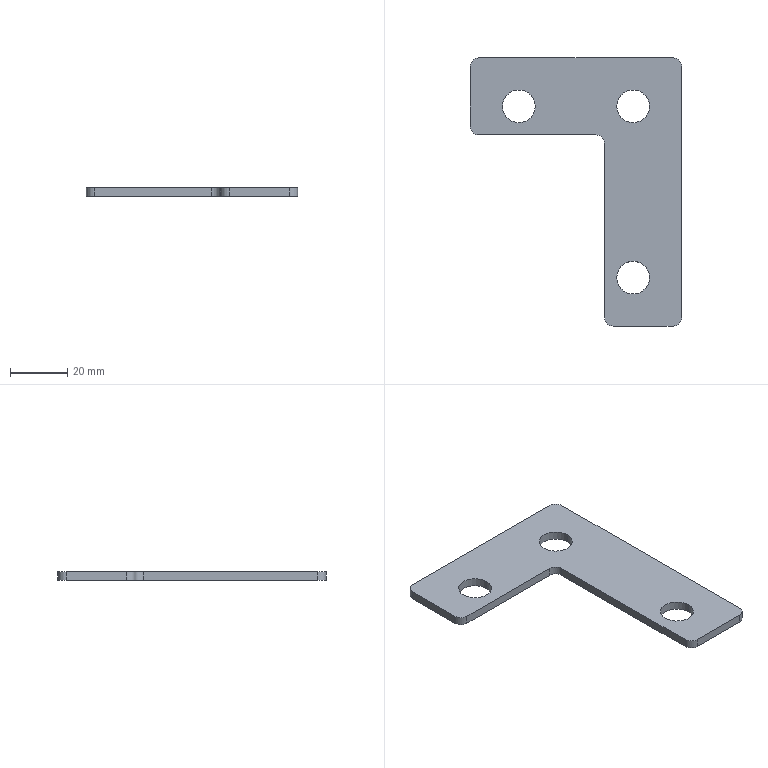Component | SolidWorks | MirrorTopBeamAssembly-2_MirrorTopBeamConnectionPlate-1 | 1 solid | 20 faces | box 74 x 94 x 3 mm | volume 10463 mm3 | cylinder 12 | plane 8 | commonest cylinder face diameters 11.5 x6 6 x6
STEP:
#1=COLOUR_RGB('',0.7922,0.8196,0.9333);
#2=FILL_AREA_STYLE_COLOUR('',#1);
#3=FILL_AREA_STYLE('',(#2));
#4=SURFACE_STYLE_FILL_AREA(#3);
#5=SURFACE_SIDE_STYLE('',(#4));
#6=SURFACE_STYLE_USAGE(.BOTH.,#5);
#7=PRESENTATION_STYLE_ASSIGNMENT((#6));
#8=CARTESIAN_POINT('',(27.442,68.39,-21.22));
#9=VERTEX_POINT('',#8);
#10=CARTESIAN_POINT('',(27.895,68.39,-21.22));
#11=VERTEX_POINT('',#10);
#12=CARTESIAN_POINT('',(27.669,68.39,-21.22));
#13=DIRECTION('',(0.,-0.,1.));
#14=DIRECTION('',(-1.,0.,0.));
#15=AXIS2_PLACEMENT_3D('',#12,#13,#14);
#16=CIRCLE('',#15,0.2264);
#17=EDGE_CURVE('',#9,#11,#16,.T.);
#18=ORIENTED_EDGE('',*,*,#17,.T.);
#19=CARTESIAN_POINT('',(27.895,68.39,-21.339));
#20=VERTEX_POINT('',#19);
#21=CARTESIAN_POINT('',(27.895,68.39,-20.945));
#22=DIRECTION('',(-0.,0.,-1.));
#23=VECTOR('',#22,39.37);
#24=LINE('',#21,#23);
#25=EDGE_CURVE('',#11,#20,#24,.T.);
#26=ORIENTED_EDGE('',*,*,#25,.T.);
#27=CARTESIAN_POINT('',(27.442,68.39,-21.339));
#28=VERTEX_POINT('',#27);
#29=CARTESIAN_POINT('',(27.669,68.39,-21.339));
#30=DIRECTION('',(0.,-0.,1.));
#31=DIRECTION('',(-1.,0.,0.));
#32=AXIS2_PLACEMENT_3D('',#29,#30,#31);
#33=CIRCLE('',#32,0.2264);
#34=EDGE_CURVE('',#28,#20,#33,.T.);
#35=ORIENTED_EDGE('',*,*,#34,.F.);
#36=CARTESIAN_POINT('',(27.442,68.39,-20.945));
#37=DIRECTION('',(-0.,0.,-1.));
#38=VECTOR('',#37,39.37);
#39=LINE('',#36,#38);
#40=EDGE_CURVE('',#9,#28,#39,.T.);
#41=ORIENTED_EDGE('',*,*,#40,.F.);
#42=EDGE_LOOP('',(#18,#26,#35,#41));
#43=FACE_OUTER_BOUND('',#42,.T.);
#44=CARTESIAN_POINT('',(27.669,68.39,-20.945));
#45=DIRECTION('',(-0.,0.,-1.));
#46=DIRECTION('',(-1.,0.,0.));
#47=AXIS2_PLACEMENT_3D('',#44,#45,#46);
#48=CYLINDRICAL_SURFACE('',#47,0.2264);
#49=ADVANCED_FACE('',(#43),#48,.F.);
#50=CARTESIAN_POINT('',(25.867,70.752,-21.22));
#51=VERTEX_POINT('',#50);
#52=CARTESIAN_POINT('',(26.32,70.752,-21.22));
#53=VERTEX_POINT('',#52);
#54=CARTESIAN_POINT('',(26.094,70.752,-21.22));
#55=DIRECTION('',(0.,-0.,1.));
#56=DIRECTION('',(-1.,0.,0.));
#57=AXIS2_PLACEMENT_3D('',#54,#55,#56);
#58=CIRCLE('',#57,0.2264);
#59=EDGE_CURVE('',#51,#53,#58,.T.);
#60=ORIENTED_EDGE('',*,*,#59,.T.);
#61=CARTESIAN_POINT('',(26.32,70.752,-21.339));
#62=VERTEX_POINT('',#61);
#63=CARTESIAN_POINT('',(26.32,70.752,-20.945));
#64=DIRECTION('',(-0.,0.,-1.));
#65=VECTOR('',#64,39.37);
#66=LINE('',#63,#65);
#67=EDGE_CURVE('',#53,#62,#66,.T.);
#68=ORIENTED_EDGE('',*,*,#67,.T.);
#69=CARTESIAN_POINT('',(25.867,70.752,-21.339));
#70=VERTEX_POINT('',#69);
#71=CARTESIAN_POINT('',(26.094,70.752,-21.339));
#72=DIRECTION('',(0.,-0.,1.));
#73=DIRECTION('',(-1.,0.,0.));
#74=AXIS2_PLACEMENT_3D('',#71,#72,#73);
#75=CIRCLE('',#74,0.2264);
#76=EDGE_CURVE('',#70,#62,#75,.T.);
#77=ORIENTED_EDGE('',*,*,#76,.F.);
#78=CARTESIAN_POINT('',(25.867,70.752,-20.945));
#79=DIRECTION('',(-0.,0.,-1.));
#80=VECTOR('',#79,39.37);
#81=LINE('',#78,#80);
#82=EDGE_CURVE('',#51,#70,#81,.T.);
#83=ORIENTED_EDGE('',*,*,#82,.F.);
#84=EDGE_LOOP('',(#60,#68,#77,#83));
#85=FACE_OUTER_BOUND('',#84,.T.);
#86=CARTESIAN_POINT('',(26.094,70.752,-20.945));
#87=DIRECTION('',(-0.,0.,-1.));
#88=DIRECTION('',(-1.,0.,0.));
#89=AXIS2_PLACEMENT_3D('',#86,#87,#88);
#90=CYLINDRICAL_SURFACE('',#89,0.2264);
#91=ADVANCED_FACE('',(#85),#90,.F.);
#92=CARTESIAN_POINT('',(27.442,70.752,-21.22));
#93=VERTEX_POINT('',#92);
#94=CARTESIAN_POINT('',(27.895,70.752,-21.22));
#95=VERTEX_POINT('',#94);
#96=CARTESIAN_POINT('',(27.669,70.752,-21.22));
#97=DIRECTION('',(0.,-0.,1.));
#98=DIRECTION('',(-1.,0.,0.));
#99=AXIS2_PLACEMENT_3D('',#96,#97,#98);
#100=CIRCLE('',#99,0.2264);
#101=EDGE_CURVE('',#93,#95,#100,.T.);
#102=ORIENTED_EDGE('',*,*,#101,.T.);
#103=CARTESIAN_POINT('',(27.895,70.752,-21.339));
#104=VERTEX_POINT('',#103);
#105=CARTESIAN_POINT('',(27.895,70.752,-20.945));
#106=DIRECTION('',(-0.,0.,-1.));
#107=VECTOR('',#106,39.37);
#108=LINE('',#105,#107);
#109=EDGE_CURVE('',#95,#104,#108,.T.);
#110=ORIENTED_EDGE('',*,*,#109,.T.);
#111=CARTESIAN_POINT('',(27.442,70.752,-21.339));
#112=VERTEX_POINT('',#111);
#113=CARTESIAN_POINT('',(27.669,70.752,-21.339));
#114=DIRECTION('',(0.,-0.,1.));
#115=DIRECTION('',(-1.,0.,0.));
#116=AXIS2_PLACEMENT_3D('',#113,#114,#115);
#117=CIRCLE('',#116,0.2264);
#118=EDGE_CURVE('',#112,#104,#117,.T.);
#119=ORIENTED_EDGE('',*,*,#118,.F.);
#120=CARTESIAN_POINT('',(27.442,70.752,-20.945));
#121=DIRECTION('',(-0.,0.,-1.));
#122=VECTOR('',#121,39.37);
#123=LINE('',#120,#122);
#124=EDGE_CURVE('',#93,#112,#123,.T.);
#125=ORIENTED_EDGE('',*,*,#124,.F.);
#126=EDGE_LOOP('',(#102,#110,#119,#125));
#127=FACE_OUTER_BOUND('',#126,.T.);
#128=CARTESIAN_POINT('',(27.669,70.752,-20.945));
#129=DIRECTION('',(-0.,0.,-1.));
#130=DIRECTION('',(-1.,0.,0.));
#131=AXIS2_PLACEMENT_3D('',#128,#129,#130);
#132=CYLINDRICAL_SURFACE('',#131,0.2264);
#133=ADVANCED_FACE('',(#127),#132,.F.);
#134=CARTESIAN_POINT('',(28.338,67.839,-21.22));
#135=VERTEX_POINT('',#134);
#136=CARTESIAN_POINT('',(28.338,71.303,-21.22));
#137=VERTEX_POINT('',#136);
#138=CARTESIAN_POINT('',(28.338,67.72,-21.22));
#139=DIRECTION('',(-0.,1.,0.));
#140=VECTOR('',#139,39.37);
#141=LINE('',#138,#140);
#142=EDGE_CURVE('',#135,#137,#141,.T.);
#143=ORIENTED_EDGE('',*,*,#142,.F.);
#144=CARTESIAN_POINT('',(28.338,67.839,-21.339));
#145=VERTEX_POINT('',#144);
#146=CARTESIAN_POINT('',(28.338,67.839,-21.22));
#147=DIRECTION('',(0.,-0.,1.));
#148=VECTOR('',#147,39.37);
#149=LINE('',#146,#148);
#150=EDGE_CURVE('',#145,#135,#149,.T.);
#151=ORIENTED_EDGE('',*,*,#150,.F.);
#152=CARTESIAN_POINT('',(28.338,71.303,-21.339));
#153=VERTEX_POINT('',#152);
#154=CARTESIAN_POINT('',(28.338,67.72,-21.339));
#155=DIRECTION('',(-0.,1.,0.));
#156=VECTOR('',#155,39.37);
#157=LINE('',#154,#156);
#158=EDGE_CURVE('',#145,#153,#157,.T.);
#159=ORIENTED_EDGE('',*,*,#158,.T.);
#160=CARTESIAN_POINT('',(28.338,71.303,-21.22));
#161=DIRECTION('',(-0.,0.,-1.));
#162=VECTOR('',#161,39.37);
#163=LINE('',#160,#162);
#164=EDGE_CURVE('',#137,#153,#163,.T.);
#165=ORIENTED_EDGE('',*,*,#164,.F.);
#166=EDGE_LOOP('',(#143,#151,#159,#165));
#167=FACE_OUTER_BOUND('',#166,.T.);
#168=CARTESIAN_POINT('',(28.338,67.72,-21.22));
#169=DIRECTION('',(1.,0.,-0.));
#170=DIRECTION('',(-0.,1.,0.));
#171=AXIS2_PLACEMENT_3D('',#168,#169,#170);
#172=PLANE('',#171);
#173=ADVANCED_FACE('',(#167),#172,.T.);
#174=CARTESIAN_POINT('',(27.393,67.72,-21.339));
#175=VERTEX_POINT('',#174);
#176=CARTESIAN_POINT('',(28.22,67.72,-21.339));
#177=VERTEX_POINT('',#176);
#178=CARTESIAN_POINT('',(27.275,67.72,-21.339));
#179=DIRECTION('',(1.,0.,-0.));
#180=VECTOR('',#179,39.37);
#181=LINE('',#178,#180);
#182=EDGE_CURVE('',#175,#177,#181,.T.);
#183=ORIENTED_EDGE('',*,*,#182,.T.);
#184=CARTESIAN_POINT('',(28.22,67.72,-21.22));
#185=VERTEX_POINT('',#184);
#186=CARTESIAN_POINT('',(28.22,67.72,-21.22));
#187=DIRECTION('',(-0.,0.,-1.));
#188=VECTOR('',#187,39.37);
#189=LINE('',#186,#188);
#190=EDGE_CURVE('',#185,#177,#189,.T.);
#191=ORIENTED_EDGE('',*,*,#190,.F.);
#192=CARTESIAN_POINT('',(27.393,67.72,-21.22));
#193=VERTEX_POINT('',#192);
#194=CARTESIAN_POINT('',(27.275,67.72,-21.22));
#195=DIRECTION('',(1.,0.,-0.));
#196=VECTOR('',#195,39.37);
#197=LINE('',#194,#196);
#198=EDGE_CURVE('',#193,#185,#197,.T.);
#199=ORIENTED_EDGE('',*,*,#198,.F.);
#200=CARTESIAN_POINT('',(27.393,67.72,-21.22));
#201=DIRECTION('',(0.,-0.,1.));
#202=VECTOR('',#201,39.37);
#203=LINE('',#200,#202);
#204=EDGE_CURVE('',#175,#193,#203,.T.);
#205=ORIENTED_EDGE('',*,*,#204,.F.);
#206=EDGE_LOOP('',(#183,#191,#199,#205));
#207=FACE_OUTER_BOUND('',#206,.T.);
#208=CARTESIAN_POINT('',(27.275,67.72,-21.22));
#209=DIRECTION('',(0.,-1.,-0.));
#210=DIRECTION('',(-0.,0.,-1.));
#211=AXIS2_PLACEMENT_3D('',#208,#209,#210);
#212=PLANE('',#211);
#213=ADVANCED_FACE('',(#207),#212,.T.);
#214=CARTESIAN_POINT('',(27.275,70.24,-21.339));
#215=VERTEX_POINT('',#214);
#216=CARTESIAN_POINT('',(27.275,67.839,-21.339));
#217=VERTEX_POINT('',#216);
#218=CARTESIAN_POINT('',(27.275,70.358,-21.339));
#219=DIRECTION('',(0.,-1.,-0.));
#220=VECTOR('',#219,39.37);
#221=LINE('',#218,#220);
#222=EDGE_CURVE('',#215,#217,#221,.T.);
#223=ORIENTED_EDGE('',*,*,#222,.T.);
#224=CARTESIAN_POINT('',(27.275,67.839,-21.22));
#225=VERTEX_POINT('',#224);
#226=CARTESIAN_POINT('',(27.275,67.839,-21.22));
#227=DIRECTION('',(-0.,0.,-1.));
#228=VECTOR('',#227,39.37);
#229=LINE('',#226,#228);
#230=EDGE_CURVE('',#225,#217,#229,.T.);
#231=ORIENTED_EDGE('',*,*,#230,.F.);
#232=CARTESIAN_POINT('',(27.275,70.24,-21.22));
#233=VERTEX_POINT('',#232);
#234=CARTESIAN_POINT('',(27.275,70.358,-21.22));
#235=DIRECTION('',(0.,-1.,-0.));
#236=VECTOR('',#235,39.37);
#237=LINE('',#234,#236);
#238=EDGE_CURVE('',#233,#225,#237,.T.);
#239=ORIENTED_EDGE('',*,*,#238,.F.);
#240=CARTESIAN_POINT('',(27.275,70.24,-21.22));
#241=DIRECTION('',(0.,-0.,1.));
#242=VECTOR('',#241,39.37);
#243=LINE('',#240,#242);
#244=EDGE_CURVE('',#215,#233,#243,.T.);
#245=ORIENTED_EDGE('',*,*,#244,.F.);
#246=EDGE_LOOP('',(#223,#231,#239,#245));
#247=FACE_OUTER_BOUND('',#246,.T.);
#248=CARTESIAN_POINT('',(27.275,70.358,-21.22));
#249=DIRECTION('',(-1.,-0.,0.));
#250=DIRECTION('',(0.,-0.,1.));
#251=AXIS2_PLACEMENT_3D('',#248,#249,#250);
#252=PLANE('',#251);
#253=ADVANCED_FACE('',(#247),#252,.T.);
#254=CARTESIAN_POINT('',(25.543,70.358,-21.22));
#255=VERTEX_POINT('',#254);
#256=CARTESIAN_POINT('',(27.157,70.358,-21.22));
#257=VERTEX_POINT('',#256);
#258=CARTESIAN_POINT('',(25.424,70.358,-21.22));
#259=DIRECTION('',(1.,0.,-0.));
#260=VECTOR('',#259,39.37);
#261=LINE('',#258,#260);
#262=EDGE_CURVE('',#255,#257,#261,.T.);
#263=ORIENTED_EDGE('',*,*,#262,.F.);
#264=CARTESIAN_POINT('',(25.543,70.358,-21.339));
#265=VERTEX_POINT('',#264);
#266=CARTESIAN_POINT('',(25.543,70.358,-21.22));
#267=DIRECTION('',(0.,-0.,1.));
#268=VECTOR('',#267,39.37);
#269=LINE('',#266,#268);
#270=EDGE_CURVE('',#265,#255,#269,.T.);
#271=ORIENTED_EDGE('',*,*,#270,.F.);
#272=CARTESIAN_POINT('',(27.157,70.358,-21.339));
#273=VERTEX_POINT('',#272);
#274=CARTESIAN_POINT('',(25.424,70.358,-21.339));
#275=DIRECTION('',(1.,0.,-0.));
#276=VECTOR('',#275,39.37);
#277=LINE('',#274,#276);
#278=EDGE_CURVE('',#265,#273,#277,.T.);
#279=ORIENTED_EDGE('',*,*,#278,.T.);
#280=CARTESIAN_POINT('',(27.157,70.358,-21.339));
#281=DIRECTION('',(-0.,0.,-1.));
#282=VECTOR('',#281,39.37);
#283=LINE('',#280,#282);
#284=EDGE_CURVE('',#257,#273,#283,.T.);
#285=ORIENTED_EDGE('',*,*,#284,.F.);
#286=EDGE_LOOP('',(#263,#271,#279,#285));
#287=FACE_OUTER_BOUND('',#286,.T.);
#288=CARTESIAN_POINT('',(25.424,70.358,-21.22));
#289=DIRECTION('',(0.,-1.,-0.));
#290=DIRECTION('',(1.,0.,-0.));
#291=AXIS2_PLACEMENT_3D('',#288,#289,#290);
#292=PLANE('',#291);
#293=ADVANCED_FACE('',(#287),#292,.T.);
#294=CARTESIAN_POINT('',(25.424,71.303,-21.339));
#295=VERTEX_POINT('',#294);
#296=CARTESIAN_POINT('',(25.424,70.476,-21.339));
#297=VERTEX_POINT('',#296);
#298=CARTESIAN_POINT('',(25.424,71.421,-21.339));
#299=DIRECTION('',(0.,-1.,-0.));
#300=VECTOR('',#299,39.37);
#301=LINE('',#298,#300);
#302=EDGE_CURVE('',#295,#297,#301,.T.);
#303=ORIENTED_EDGE('',*,*,#302,.T.);
#304=CARTESIAN_POINT('',(25.424,70.476,-21.22));
#305=VERTEX_POINT('',#304);
#306=CARTESIAN_POINT('',(25.424,70.476,-21.22));
#307=DIRECTION('',(-0.,0.,-1.));
#308=VECTOR('',#307,39.37);
#309=LINE('',#306,#308);
#310=EDGE_CURVE('',#305,#297,#309,.T.);
#311=ORIENTED_EDGE('',*,*,#310,.F.);
#312=CARTESIAN_POINT('',(25.424,71.303,-21.22));
#313=VERTEX_POINT('',#312);
#314=CARTESIAN_POINT('',(25.424,71.421,-21.22));
#315=DIRECTION('',(0.,-1.,-0.));
#316=VECTOR('',#315,39.37);
#317=LINE('',#314,#316);
#318=EDGE_CURVE('',#313,#305,#317,.T.);
#319=ORIENTED_EDGE('',*,*,#318,.F.);
#320=CARTESIAN_POINT('',(25.424,71.303,-21.22));
#321=DIRECTION('',(0.,-0.,1.));
#322=VECTOR('',#321,39.37);
#323=LINE('',#320,#322);
#324=EDGE_CURVE('',#295,#313,#323,.T.);
#325=ORIENTED_EDGE('',*,*,#324,.F.);
#326=EDGE_LOOP('',(#303,#311,#319,#325));
#327=FACE_OUTER_BOUND('',#326,.T.);
#328=CARTESIAN_POINT('',(25.424,71.421,-21.22));
#329=DIRECTION('',(-1.,-0.,0.));
#330=DIRECTION('',(0.,-0.,1.));
#331=AXIS2_PLACEMENT_3D('',#328,#329,#330);
#332=PLANE('',#331);
#333=ADVANCED_FACE('',(#327),#332,.T.);
#334=CARTESIAN_POINT('',(28.22,71.421,-21.339));
#335=VERTEX_POINT('',#334);
#336=CARTESIAN_POINT('',(25.543,71.421,-21.339));
#337=VERTEX_POINT('',#336);
#338=CARTESIAN_POINT('',(28.338,71.421,-21.339));
#339=DIRECTION('',(-1.,-0.,0.));
#340=VECTOR('',#339,39.37);
#341=LINE('',#338,#340);
#342=EDGE_CURVE('',#335,#337,#341,.T.);
#343=ORIENTED_EDGE('',*,*,#342,.T.);
#344=CARTESIAN_POINT('',(25.543,71.421,-21.22));
#345=VERTEX_POINT('',#344);
#346=CARTESIAN_POINT('',(25.543,71.421,-21.22));
#347=DIRECTION('',(-0.,0.,-1.));
#348=VECTOR('',#347,39.37);
#349=LINE('',#346,#348);
#350=EDGE_CURVE('',#345,#337,#349,.T.);
#351=ORIENTED_EDGE('',*,*,#350,.F.);
#352=CARTESIAN_POINT('',(28.22,71.421,-21.22));
#353=VERTEX_POINT('',#352);
#354=CARTESIAN_POINT('',(28.338,71.421,-21.22));
#355=DIRECTION('',(-1.,-0.,0.));
#356=VECTOR('',#355,39.37);
#357=LINE('',#354,#356);
#358=EDGE_CURVE('',#353,#345,#357,.T.);
#359=ORIENTED_EDGE('',*,*,#358,.F.);
#360=CARTESIAN_POINT('',(28.22,71.421,-21.22));
#361=DIRECTION('',(0.,-0.,1.));
#362=VECTOR('',#361,39.37);
#363=LINE('',#360,#362);
#364=EDGE_CURVE('',#335,#353,#363,.T.);
#365=ORIENTED_EDGE('',*,*,#364,.F.);
#366=EDGE_LOOP('',(#343,#351,#359,#365));
#367=FACE_OUTER_BOUND('',#366,.T.);
#368=CARTESIAN_POINT('',(28.338,71.421,-21.22));
#369=DIRECTION('',(-0.,1.,0.));
#370=DIRECTION('',(0.,-0.,1.));
#371=AXIS2_PLACEMENT_3D('',#368,#369,#370);
#372=PLANE('',#371);
#373=ADVANCED_FACE('',(#367),#372,.T.);
#374=ORIENTED_EDGE('',*,*,#17,.F.);
#375=CARTESIAN_POINT('',(27.669,68.39,-21.22));
#376=DIRECTION('',(0.,-0.,1.));
#377=DIRECTION('',(-1.,0.,0.));
#378=AXIS2_PLACEMENT_3D('',#375,#376,#377);
#379=CIRCLE('',#378,0.2264);
#380=EDGE_CURVE('',#11,#9,#379,.T.);
#381=ORIENTED_EDGE('',*,*,#380,.F.);
#382=EDGE_LOOP('',(#374,#381));
#383=FACE_BOUND('',#382,.T.);
#384=ORIENTED_EDGE('',*,*,#59,.F.);
#385=CARTESIAN_POINT('',(26.094,70.752,-21.22));
#386=DIRECTION('',(0.,-0.,1.));
#387=DIRECTION('',(-1.,0.,0.));
#388=AXIS2_PLACEMENT_3D('',#385,#386,#387);
#389=CIRCLE('',#388,0.2264);
#390=EDGE_CURVE('',#53,#51,#389,.T.);
#391=ORIENTED_EDGE('',*,*,#390,.F.);
#392=EDGE_LOOP('',(#384,#391));
#393=FACE_BOUND('',#392,.T.);
#394=ORIENTED_EDGE('',*,*,#101,.F.);
#395=CARTESIAN_POINT('',(27.669,70.752,-21.22));
#396=DIRECTION('',(0.,-0.,1.));
#397=DIRECTION('',(-1.,0.,0.));
#398=AXIS2_PLACEMENT_3D('',#395,#396,#397);
#399=CIRCLE('',#398,0.2264);
#400=EDGE_CURVE('',#95,#93,#399,.T.);
#401=ORIENTED_EDGE('',*,*,#400,.F.);
#402=EDGE_LOOP('',(#394,#401));
#403=FACE_BOUND('',#402,.T.);
#404=ORIENTED_EDGE('',*,*,#358,.T.);
#405=CARTESIAN_POINT('',(25.543,71.303,-21.22));
#406=DIRECTION('',(-0.,0.,-1.));
#407=DIRECTION('',(-1.,0.,0.));
#408=AXIS2_PLACEMENT_3D('',#405,#406,#407);
#409=CIRCLE('',#408,0.1181);
#410=EDGE_CURVE('',#313,#345,#409,.T.);
#411=ORIENTED_EDGE('',*,*,#410,.F.);
#412=ORIENTED_EDGE('',*,*,#318,.T.);
#413=CARTESIAN_POINT('',(25.543,70.476,-21.22));
#414=DIRECTION('',(-0.,0.,-1.));
#415=DIRECTION('',(-1.,0.,0.));
#416=AXIS2_PLACEMENT_3D('',#413,#414,#415);
#417=CIRCLE('',#416,0.1181);
#418=EDGE_CURVE('',#255,#305,#417,.T.);
#419=ORIENTED_EDGE('',*,*,#418,.F.);
#420=ORIENTED_EDGE('',*,*,#262,.T.);
#421=CARTESIAN_POINT('',(27.157,70.24,-21.22));
#422=DIRECTION('',(0.,-0.,1.));
#423=DIRECTION('',(-1.,0.,0.));
#424=AXIS2_PLACEMENT_3D('',#421,#422,#423);
#425=CIRCLE('',#424,0.1181);
#426=EDGE_CURVE('',#233,#257,#425,.T.);
#427=ORIENTED_EDGE('',*,*,#426,.F.);
#428=ORIENTED_EDGE('',*,*,#238,.T.);
#429=CARTESIAN_POINT('',(27.393,67.839,-21.22));
#430=DIRECTION('',(-0.,0.,-1.));
#431=DIRECTION('',(-1.,0.,0.));
#432=AXIS2_PLACEMENT_3D('',#429,#430,#431);
#433=CIRCLE('',#432,0.1181);
#434=EDGE_CURVE('',#193,#225,#433,.T.);
#435=ORIENTED_EDGE('',*,*,#434,.F.);
#436=ORIENTED_EDGE('',*,*,#198,.T.);
#437=CARTESIAN_POINT('',(28.22,67.839,-21.22));
#438=DIRECTION('',(-0.,0.,-1.));
#439=DIRECTION('',(-1.,0.,0.));
#440=AXIS2_PLACEMENT_3D('',#437,#438,#439);
#441=CIRCLE('',#440,0.1181);
#442=EDGE_CURVE('',#135,#185,#441,.T.);
#443=ORIENTED_EDGE('',*,*,#442,.F.);
#444=ORIENTED_EDGE('',*,*,#142,.T.);
#445=CARTESIAN_POINT('',(28.22,71.303,-21.22));
#446=DIRECTION('',(-0.,0.,-1.));
#447=DIRECTION('',(-1.,0.,0.));
#448=AXIS2_PLACEMENT_3D('',#445,#446,#447);
#449=CIRCLE('',#448,0.1181);
#450=EDGE_CURVE('',#353,#137,#449,.T.);
#451=ORIENTED_EDGE('',*,*,#450,.F.);
#452=EDGE_LOOP('',(#404,#411,#412,#419,#420,#427,#428,#435,#436,#443,#444,#451));
#453=FACE_OUTER_BOUND('',#452,.T.);
#454=CARTESIAN_POINT('',(28.338,71.421,-21.22));
#455=DIRECTION('',(-0.,0.,-1.));
#456=DIRECTION('',(-1.,-0.,0.));
#457=AXIS2_PLACEMENT_3D('',#454,#455,#456);
#458=PLANE('',#457);
#459=ADVANCED_FACE('',(#383,#393,#403,#453),#458,.F.);
#460=ORIENTED_EDGE('',*,*,#34,.T.);
#461=CARTESIAN_POINT('',(27.669,68.39,-21.339));
#462=DIRECTION('',(0.,-0.,1.));
#463=DIRECTION('',(-1.,0.,0.));
#464=AXIS2_PLACEMENT_3D('',#461,#462,#463);
#465=CIRCLE('',#464,0.2264);
#466=EDGE_CURVE('',#20,#28,#465,.T.);
#467=ORIENTED_EDGE('',*,*,#466,.T.);
#468=EDGE_LOOP('',(#460,#467));
#469=FACE_BOUND('',#468,.T.);
#470=ORIENTED_EDGE('',*,*,#76,.T.);
#471=CARTESIAN_POINT('',(26.094,70.752,-21.339));
#472=DIRECTION('',(0.,-0.,1.));
#473=DIRECTION('',(-1.,0.,0.));
#474=AXIS2_PLACEMENT_3D('',#471,#472,#473);
#475=CIRCLE('',#474,0.2264);
#476=EDGE_CURVE('',#62,#70,#475,.T.);
#477=ORIENTED_EDGE('',*,*,#476,.T.);
#478=EDGE_LOOP('',(#470,#477));
#479=FACE_BOUND('',#478,.T.);
#480=ORIENTED_EDGE('',*,*,#118,.T.);
#481=CARTESIAN_POINT('',(27.669,70.752,-21.339));
#482=DIRECTION('',(0.,-0.,1.));
#483=DIRECTION('',(-1.,0.,0.));
#484=AXIS2_PLACEMENT_3D('',#481,#482,#483);
#485=CIRCLE('',#484,0.2264);
#486=EDGE_CURVE('',#104,#112,#485,.T.);
#487=ORIENTED_EDGE('',*,*,#486,.T.);
#488=EDGE_LOOP('',(#480,#487));
#489=FACE_BOUND('',#488,.T.);
#490=ORIENTED_EDGE('',*,*,#158,.F.);
#491=CARTESIAN_POINT('',(28.22,67.839,-21.339));
#492=DIRECTION('',(0.,-0.,1.));
#493=DIRECTION('',(-1.,0.,0.));
#494=AXIS2_PLACEMENT_3D('',#491,#492,#493);
#495=CIRCLE('',#494,0.1181);
#496=EDGE_CURVE('',#177,#145,#495,.T.);
#497=ORIENTED_EDGE('',*,*,#496,.F.);
#498=ORIENTED_EDGE('',*,*,#182,.F.);
#499=CARTESIAN_POINT('',(27.393,67.839,-21.339));
#500=DIRECTION('',(0.,-0.,1.));
#501=DIRECTION('',(-1.,0.,0.));
#502=AXIS2_PLACEMENT_3D('',#499,#500,#501);
#503=CIRCLE('',#502,0.1181);
#504=EDGE_CURVE('',#217,#175,#503,.T.);
#505=ORIENTED_EDGE('',*,*,#504,.F.);
#506=ORIENTED_EDGE('',*,*,#222,.F.);
#507=CARTESIAN_POINT('',(27.157,70.24,-21.339));
#508=DIRECTION('',(-0.,0.,-1.));
#509=DIRECTION('',(-1.,0.,0.));
#510=AXIS2_PLACEMENT_3D('',#507,#508,#509);
#511=CIRCLE('',#510,0.1181);
#512=EDGE_CURVE('',#273,#215,#511,.T.);
#513=ORIENTED_EDGE('',*,*,#512,.F.);
#514=ORIENTED_EDGE('',*,*,#278,.F.);
#515=CARTESIAN_POINT('',(25.543,70.476,-21.339));
#516=DIRECTION('',(0.,-0.,1.));
#517=DIRECTION('',(-1.,0.,0.));
#518=AXIS2_PLACEMENT_3D('',#515,#516,#517);
#519=CIRCLE('',#518,0.1181);
#520=EDGE_CURVE('',#297,#265,#519,.T.);
#521=ORIENTED_EDGE('',*,*,#520,.F.);
#522=ORIENTED_EDGE('',*,*,#302,.F.);
#523=CARTESIAN_POINT('',(25.543,71.303,-21.339));
#524=DIRECTION('',(0.,-0.,1.));
#525=DIRECTION('',(-1.,0.,0.));
#526=AXIS2_PLACEMENT_3D('',#523,#524,#525);
#527=CIRCLE('',#526,0.1181);
#528=EDGE_CURVE('',#337,#295,#527,.T.);
#529=ORIENTED_EDGE('',*,*,#528,.F.);
#530=ORIENTED_EDGE('',*,*,#342,.F.);
#531=CARTESIAN_POINT('',(28.22,71.303,-21.339));
#532=DIRECTION('',(0.,-0.,1.));
#533=DIRECTION('',(-1.,0.,0.));
#534=AXIS2_PLACEMENT_3D('',#531,#532,#533);
#535=CIRCLE('',#534,0.1181);
#536=EDGE_CURVE('',#153,#335,#535,.T.);
#537=ORIENTED_EDGE('',*,*,#536,.F.);
#538=EDGE_LOOP('',(#490,#497,#498,#505,#506,#513,#514,#521,#522,#529,#530,#537));
#539=FACE_OUTER_BOUND('',#538,.T.);
#540=CARTESIAN_POINT('',(28.338,71.421,-21.339));
#541=DIRECTION('',(-0.,0.,-1.));
#542=DIRECTION('',(-1.,-0.,0.));
#543=AXIS2_PLACEMENT_3D('',#540,#541,#542);
#544=PLANE('',#543);
#545=ADVANCED_FACE('',(#469,#479,#489,#539),#544,.T.);
#546=ORIENTED_EDGE('',*,*,#426,.T.);
#547=ORIENTED_EDGE('',*,*,#284,.T.);
#548=ORIENTED_EDGE('',*,*,#512,.T.);
#549=ORIENTED_EDGE('',*,*,#244,.T.);
#550=EDGE_LOOP('',(#546,#547,#548,#549));
#551=FACE_OUTER_BOUND('',#550,.T.);
#552=CARTESIAN_POINT('',(27.157,70.24,-21.22));
#553=DIRECTION('',(0.,-0.,1.));
#554=DIRECTION('',(1.,0.,0.));
#555=AXIS2_PLACEMENT_3D('',#552,#553,#554);
#556=CYLINDRICAL_SURFACE('',#555,0.1181);
#557=ADVANCED_FACE('',(#551),#556,.F.);
#558=ORIENTED_EDGE('',*,*,#450,.T.);
#559=ORIENTED_EDGE('',*,*,#164,.T.);
#560=ORIENTED_EDGE('',*,*,#536,.T.);
#561=ORIENTED_EDGE('',*,*,#364,.T.);
#562=EDGE_LOOP('',(#558,#559,#560,#561));
#563=FACE_OUTER_BOUND('',#562,.T.);
#564=CARTESIAN_POINT('',(28.22,71.303,-21.22));
#565=DIRECTION('',(-0.,0.,-1.));
#566=DIRECTION('',(-1.,0.,0.));
#567=AXIS2_PLACEMENT_3D('',#564,#565,#566);
#568=CYLINDRICAL_SURFACE('',#567,0.1181);
#569=ADVANCED_FACE('',(#563),#568,.T.);
#570=ORIENTED_EDGE('',*,*,#410,.T.);
#571=ORIENTED_EDGE('',*,*,#350,.T.);
#572=ORIENTED_EDGE('',*,*,#528,.T.);
#573=ORIENTED_EDGE('',*,*,#324,.T.);
#574=EDGE_LOOP('',(#570,#571,#572,#573));
#575=FACE_OUTER_BOUND('',#574,.T.);
#576=CARTESIAN_POINT('',(25.543,71.303,-21.22));
#577=DIRECTION('',(-0.,0.,-1.));
#578=DIRECTION('',(-1.,0.,0.));
#579=AXIS2_PLACEMENT_3D('',#576,#577,#578);
#580=CYLINDRICAL_SURFACE('',#579,0.1181);
#581=ADVANCED_FACE('',(#575),#580,.T.);
#582=ORIENTED_EDGE('',*,*,#418,.T.);
#583=ORIENTED_EDGE('',*,*,#310,.T.);
#584=ORIENTED_EDGE('',*,*,#520,.T.);
#585=ORIENTED_EDGE('',*,*,#270,.T.);
#586=EDGE_LOOP('',(#582,#583,#584,#585));
#587=FACE_OUTER_BOUND('',#586,.T.);
#588=CARTESIAN_POINT('',(25.543,70.476,-21.22));
#589=DIRECTION('',(-0.,0.,-1.));
#590=DIRECTION('',(-1.,0.,0.));
#591=AXIS2_PLACEMENT_3D('',#588,#589,#590);
#592=CYLINDRICAL_SURFACE('',#591,0.1181);
#593=ADVANCED_FACE('',(#587),#592,.T.);
#594=ORIENTED_EDGE('',*,*,#434,.T.);
#595=ORIENTED_EDGE('',*,*,#230,.T.);
#596=ORIENTED_EDGE('',*,*,#504,.T.);
#597=ORIENTED_EDGE('',*,*,#204,.T.);
#598=EDGE_LOOP('',(#594,#595,#596,#597));
#599=FACE_OUTER_BOUND('',#598,.T.);
#600=CARTESIAN_POINT('',(27.393,67.839,-21.22));
#601=DIRECTION('',(-0.,0.,-1.));
#602=DIRECTION('',(-1.,0.,0.));
#603=AXIS2_PLACEMENT_3D('',#600,#601,#602);
#604=CYLINDRICAL_SURFACE('',#603,0.1181);
#605=ADVANCED_FACE('',(#599),#604,.T.);
#606=ORIENTED_EDGE('',*,*,#442,.T.);
#607=ORIENTED_EDGE('',*,*,#190,.T.);
#608=ORIENTED_EDGE('',*,*,#496,.T.);
#609=ORIENTED_EDGE('',*,*,#150,.T.);
#610=EDGE_LOOP('',(#606,#607,#608,#609));
#611=FACE_OUTER_BOUND('',#610,.T.);
#612=CARTESIAN_POINT('',(28.22,67.839,-21.22));
#613=DIRECTION('',(-0.,0.,-1.));
#614=DIRECTION('',(-1.,0.,0.));
#615=AXIS2_PLACEMENT_3D('',#612,#613,#614);
#616=CYLINDRICAL_SURFACE('',#615,0.1181);
#617=ADVANCED_FACE('',(#611),#616,.T.);
#618=ORIENTED_EDGE('',*,*,#109,.F.);
#619=ORIENTED_EDGE('',*,*,#400,.T.);
#620=ORIENTED_EDGE('',*,*,#124,.T.);
#621=ORIENTED_EDGE('',*,*,#486,.F.);
#622=EDGE_LOOP('',(#618,#619,#620,#621));
#623=FACE_OUTER_BOUND('',#622,.T.);
#624=CARTESIAN_POINT('',(27.669,70.752,-20.945));
#625=DIRECTION('',(-0.,0.,-1.));
#626=DIRECTION('',(-1.,0.,0.));
#627=AXIS2_PLACEMENT_3D('',#624,#625,#626);
#628=CYLINDRICAL_SURFACE('',#627,0.2264);
#629=ADVANCED_FACE('',(#623),#628,.F.);
#630=ORIENTED_EDGE('',*,*,#67,.F.);
#631=ORIENTED_EDGE('',*,*,#390,.T.);
#632=ORIENTED_EDGE('',*,*,#82,.T.);
#633=ORIENTED_EDGE('',*,*,#476,.F.);
#634=EDGE_LOOP('',(#630,#631,#632,#633));
#635=FACE_OUTER_BOUND('',#634,.T.);
#636=CARTESIAN_POINT('',(26.094,70.752,-20.945));
#637=DIRECTION('',(-0.,0.,-1.));
#638=DIRECTION('',(-1.,0.,0.));
#639=AXIS2_PLACEMENT_3D('',#636,#637,#638);
#640=CYLINDRICAL_SURFACE('',#639,0.2264);
#641=ADVANCED_FACE('',(#635),#640,.F.);
#642=ORIENTED_EDGE('',*,*,#25,.F.);
#643=ORIENTED_EDGE('',*,*,#380,.T.);
#644=ORIENTED_EDGE('',*,*,#40,.T.);
#645=ORIENTED_EDGE('',*,*,#466,.F.);
#646=EDGE_LOOP('',(#642,#643,#644,#645));
#647=FACE_OUTER_BOUND('',#646,.T.);
#648=CARTESIAN_POINT('',(27.669,68.39,-20.945));
#649=DIRECTION('',(-0.,0.,-1.));
#650=DIRECTION('',(-1.,0.,0.));
#651=AXIS2_PLACEMENT_3D('',#648,#649,#650);
#652=CYLINDRICAL_SURFACE('',#651,0.2264);
#653=ADVANCED_FACE('',(#647),#652,.F.);
#654=CLOSED_SHELL('',(#49,#91,#133,#173,#213,#253,#293,#333,#373,#459,#545,#557,#569,#581,#593,#605,#617,#629,#641,#653));
#655=MANIFOLD_SOLID_BREP('',#654);
#656=STYLED_ITEM('',(#7),#655);
#657=(LENGTH_UNIT()NAMED_UNIT(*)SI_UNIT($,.METRE.));
#658=LENGTH_MEASURE_WITH_UNIT(LENGTH_MEASURE(0.0254),#657);
#659=DIMENSIONAL_EXPONENTS(1.,0.,0.,0.,0.,0.,0.);
#660=(CONVERSION_BASED_UNIT('',#658)LENGTH_UNIT()NAMED_UNIT(#659));
#661=UNCERTAINTY_MEASURE_WITH_UNIT(LENGTH_MEASURE(0.00001),#660,'','');
#662=(NAMED_UNIT(*)PLANE_ANGLE_UNIT()SI_UNIT($,.RADIAN.));
#663=(NAMED_UNIT(*)SI_UNIT($,.STERADIAN.)SOLID_ANGLE_UNIT());
#664=(GEOMETRIC_REPRESENTATION_CONTEXT(3)GLOBAL_UNCERTAINTY_ASSIGNED_CONTEXT((#661))GLOBAL_UNIT_ASSIGNED_CONTEXT((#660,#662,#663))REPRESENTATION_CONTEXT('',''));
#665=MECHANICAL_DESIGN_GEOMETRIC_PRESENTATION_REPRESENTATION('',(#656),#664);
#666=CARTESIAN_POINT('',(0.,0.,0.));
#667=DIRECTION('',(0.,0.,1.));
#668=DIRECTION('',(1.,0.,0.));
#669=AXIS2_PLACEMENT_3D('',#666,#667,#668);
#670=(LENGTH_UNIT()NAMED_UNIT(*)SI_UNIT($,.METRE.));
#671=LENGTH_MEASURE_WITH_UNIT(LENGTH_MEASURE(0.0254),#670);
#672=DIMENSIONAL_EXPONENTS(1.,0.,0.,0.,0.,0.,0.);
#673=(CONVERSION_BASED_UNIT('',#671)LENGTH_UNIT()NAMED_UNIT(#672));
#674=UNCERTAINTY_MEASURE_WITH_UNIT(LENGTH_MEASURE(0.00001),#673,'','');
#675=(NAMED_UNIT(*)PLANE_ANGLE_UNIT()SI_UNIT($,.RADIAN.));
#676=(NAMED_UNIT(*)SI_UNIT($,.STERADIAN.)SOLID_ANGLE_UNIT());
#677=(GEOMETRIC_REPRESENTATION_CONTEXT(3)GLOBAL_UNCERTAINTY_ASSIGNED_CONTEXT((#674))GLOBAL_UNIT_ASSIGNED_CONTEXT((#673,#675,#676))REPRESENTATION_CONTEXT('',''));
#678=ADVANCED_BREP_SHAPE_REPRESENTATION('',(#655,#669),#677);
#679=PRESENTATION_LAYER_ASSIGNMENT('','',(#656));